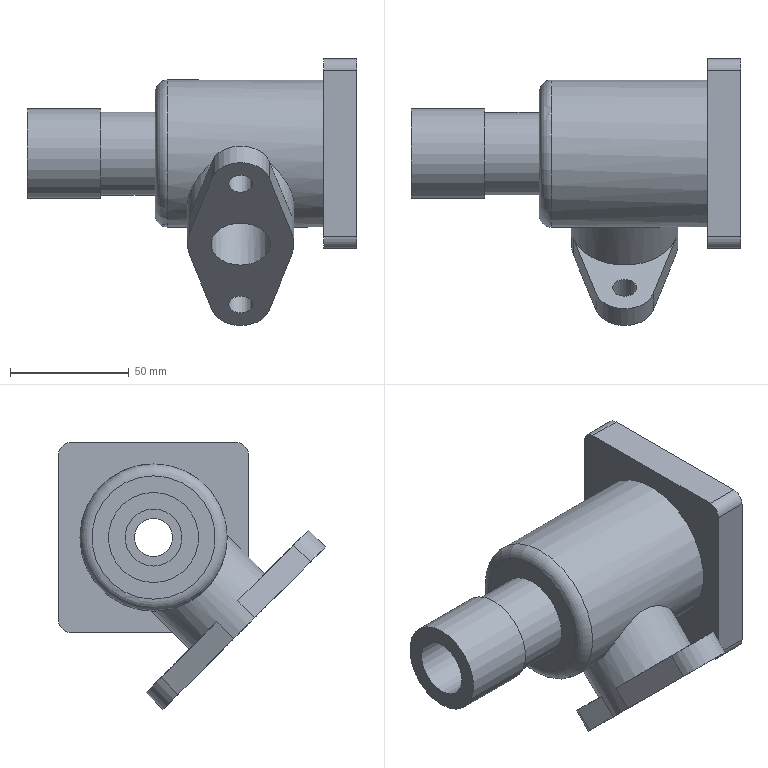Component | NX | VALVE_BODY | 1 solid | 49 faces | volume 189048 mm3 | cylinder 22 | plane 19 | cone 4 | torus 3 | spline 1 | commonest cylinder face diameters 10 x6 6 x4 25 x3 56 x1 62 x1 24 x1 16 x1 50 x1